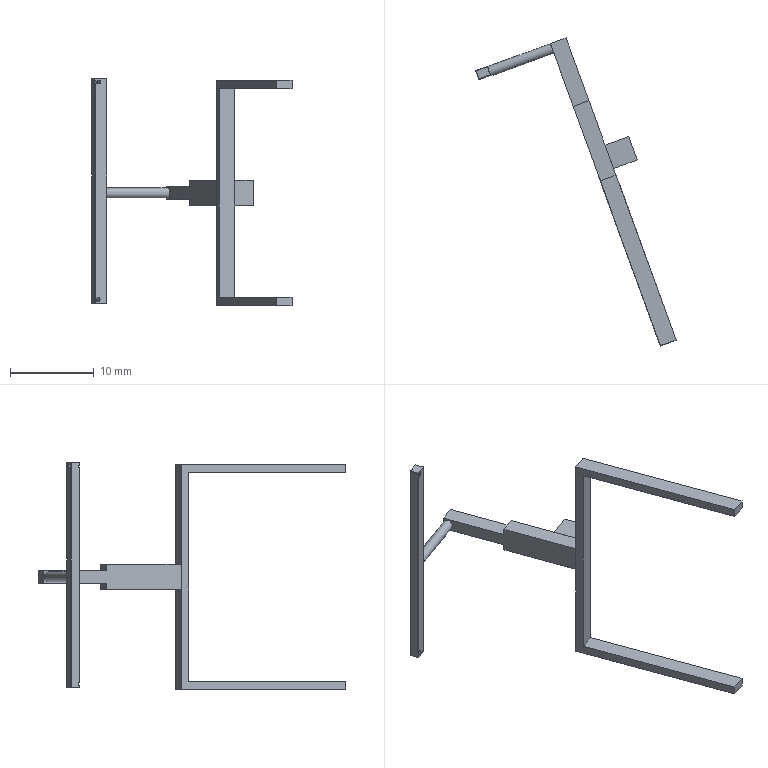Component | NX | MODEL7 | 5 solids | 82 faces | volume 295 mm3 | plane 42 | cylinder 30 | sphere 10 | commonest cylinder face diameters 0.1 x14 0.086 x13 0.501 x1 0.452 x1 1.2 x1